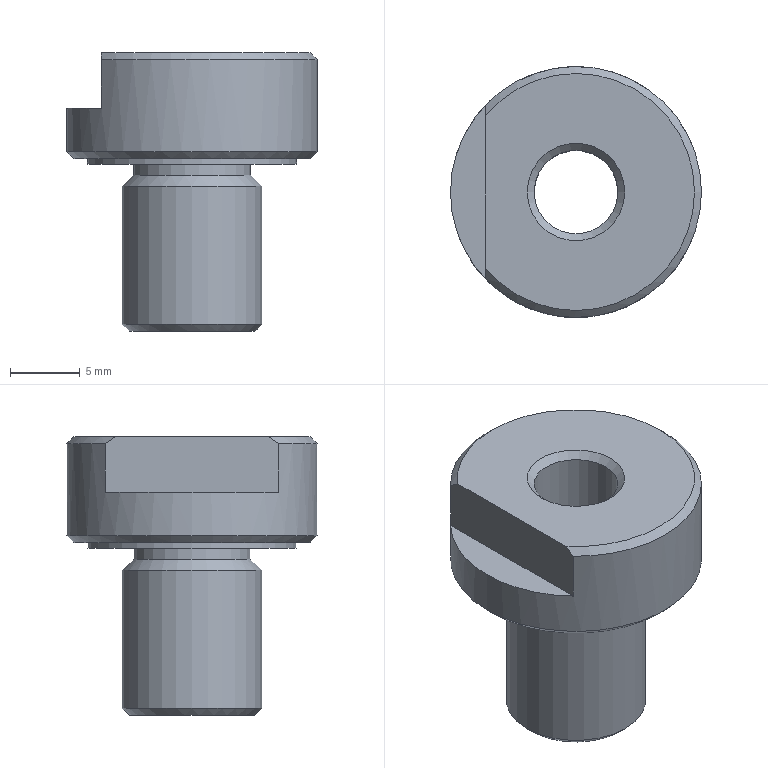Component | NX | DRILL_BUSHING | 1 solid | 17 faces | box 18 x 18 x 20 mm | volume 2247 mm3 | plane 6 | cone 6 | cylinder 5 | commonest cylinder face diameters 18 x1 15 x1 8.4 x1 10 x1 6 x1
STEP:
#1=CARTESIAN_POINT('',(0.,0.,0.));
#2=DIRECTION('',(0.,0.,1.));
#3=DIRECTION('',(1.,0.,0.));
#4=AXIS2_PLACEMENT_3D('',#1,#2,#3);
#5=CARTESIAN_POINT('',(15.5,100.638,-196.5));
#6=VERTEX_POINT('',#5);
#7=CARTESIAN_POINT('',(12.,100.638,-196.5));
#8=DIRECTION('',(0.,0.,-1.));
#9=DIRECTION('',(1.,0.,0.));
#10=AXIS2_PLACEMENT_3D('',#7,#8,#9);
#11=CIRCLE('',#10,3.5);
#12=CARTESIAN_POINT('',(12.,104.138,-196.5));
#13=DIRECTION('',(0.,0.,-1.));
#14=DIRECTION('',(1.,0.,0.));
#15=AXIS2_PLACEMENT_3D('',#12,#13,#14);
#16=PLANE('',#15);
#17=CARTESIAN_POINT('',(0.,3.5));
#18=DIRECTION('',(1.,0.));
#19=AXIS2_PLACEMENT_2D('',#17,#18);
#20=CIRCLE('',#19,3.5);
#21=(GEOMETRIC_REPRESENTATION_CONTEXT(2)PARAMETRIC_REPRESENTATION_CONTEXT()REPRESENTATION_CONTEXT('',''));
#22=DEFINITIONAL_REPRESENTATION('',(#20),#21);
#23=PCURVE('',#16,#22);
#24=CARTESIAN_POINT('',(12.,100.638,-197.));
#25=DIRECTION('',(0.,0.,1.));
#26=DIRECTION('',(-1.,0.,0.));
#27=AXIS2_PLACEMENT_3D('',#24,#25,#26);
#28=CONICAL_SURFACE('',#27,3.,0.7854);
#29=CARTESIAN_POINT('',(9.425,0.5));
#30=DIRECTION('',(-1.,0.));
#31=VECTOR('',#30,1.);
#32=LINE('',#29,#31);
#33=(GEOMETRIC_REPRESENTATION_CONTEXT(2)PARAMETRIC_REPRESENTATION_CONTEXT()REPRESENTATION_CONTEXT('',''));
#34=DEFINITIONAL_REPRESENTATION('',(#32),#33);
#35=PCURVE('',#28,#34);
#36=SURFACE_CURVE('',#11,(#23,#35),.PCURVE_S1.);
#37=EDGE_CURVE('',#6,#6,#36,.T.);
#38=ORIENTED_EDGE('',*,*,#37,.T.);
#39=EDGE_LOOP('',(#38));
#40=FACE_BOUND('',#39,.T.);
#41=CARTESIAN_POINT('',(5.5,95.161,-196.5));
#42=VERTEX_POINT('',#41);
#43=CARTESIAN_POINT('',(5.5,106.116,-196.5));
#44=VERTEX_POINT('',#43);
#45=CARTESIAN_POINT('',(5.5,88.638,-196.5));
#46=DIRECTION('',(-0.,1.,0.));
#47=VECTOR('',#46,1.);
#48=LINE('',#45,#47);
#49=CARTESIAN_POINT('',(-6.5,15.5));
#50=DIRECTION('',(-0.,-1.));
#51=VECTOR('',#50,1.);
#52=LINE('',#49,#51);
#53=(GEOMETRIC_REPRESENTATION_CONTEXT(2)PARAMETRIC_REPRESENTATION_CONTEXT()REPRESENTATION_CONTEXT('',''));
#54=DEFINITIONAL_REPRESENTATION('',(#52),#53);
#55=PCURVE('',#16,#54);
#56=CARTESIAN_POINT('',(5.5,88.638,-200.5));
#57=DIRECTION('',(1.,0.,0.));
#58=DIRECTION('',(-0.,1.,0.));
#59=AXIS2_PLACEMENT_3D('',#56,#57,#58);
#60=PLANE('',#59);
#61=CARTESIAN_POINT('',(0.,4.));
#62=DIRECTION('',(1.,0.));
#63=VECTOR('',#62,1.);
#64=LINE('',#61,#63);
#65=(GEOMETRIC_REPRESENTATION_CONTEXT(2)PARAMETRIC_REPRESENTATION_CONTEXT()REPRESENTATION_CONTEXT('',''));
#66=DEFINITIONAL_REPRESENTATION('',(#64),#65);
#67=PCURVE('',#60,#66);
#68=SURFACE_CURVE('',#48,(#55,#67),.PCURVE_S1.);
#69=EDGE_CURVE('',#42,#44,#68,.T.);
#70=ORIENTED_EDGE('',*,*,#69,.F.);
#71=CARTESIAN_POINT('',(12.,100.638,-196.5));
#72=DIRECTION('',(0.,0.,-1.));
#73=DIRECTION('',(1.,0.,0.));
#74=AXIS2_PLACEMENT_3D('',#71,#72,#73);
#75=CIRCLE('',#74,8.5);
#76=CARTESIAN_POINT('',(0.,3.5));
#77=DIRECTION('',(1.,0.));
#78=AXIS2_PLACEMENT_2D('',#76,#77);
#79=CIRCLE('',#78,8.5);
#80=(GEOMETRIC_REPRESENTATION_CONTEXT(2)PARAMETRIC_REPRESENTATION_CONTEXT()REPRESENTATION_CONTEXT('',''));
#81=DEFINITIONAL_REPRESENTATION('',(#79),#80);
#82=PCURVE('',#16,#81);
#83=CARTESIAN_POINT('',(12.,100.638,-196.5));
#84=DIRECTION('',(0.,0.,-1.));
#85=DIRECTION('',(1.,0.,0.));
#86=AXIS2_PLACEMENT_3D('',#83,#84,#85);
#87=CONICAL_SURFACE('',#86,8.5,0.7854);
#88=CARTESIAN_POINT('',(-6.283,0.));
#89=DIRECTION('',(1.,-0.));
#90=VECTOR('',#89,1.);
#91=LINE('',#88,#90);
#92=(GEOMETRIC_REPRESENTATION_CONTEXT(2)PARAMETRIC_REPRESENTATION_CONTEXT()REPRESENTATION_CONTEXT('',''));
#93=DEFINITIONAL_REPRESENTATION('',(#91),#92);
#94=PCURVE('',#87,#93);
#95=SURFACE_CURVE('',#75,(#82,#94),.PCURVE_S1.);
#96=EDGE_CURVE('',#44,#42,#95,.T.);
#97=ORIENTED_EDGE('',*,*,#96,.F.);
#98=EDGE_LOOP('',(#70,#97));
#99=FACE_BOUND('',#98,.T.);
#100=ADVANCED_FACE('',(#40,#99),#16,.F.);
#101=CARTESIAN_POINT('',(5.5,106.863,-197.));
#102=VERTEX_POINT('',#101);
#103=CARTESIAN_POINT('',(21.,100.638,-197.));
#104=VERTEX_POINT('',#103);
#105=CARTESIAN_POINT('',(12.,100.638,-197.));
#106=DIRECTION('',(0.,0.,-1.));
#107=DIRECTION('',(1.,0.,0.));
#108=AXIS2_PLACEMENT_3D('',#105,#106,#107);
#109=CIRCLE('',#108,9.);
#110=CARTESIAN_POINT('',(12.,100.638,-216.5));
#111=DIRECTION('',(0.,0.,-1.));
#112=DIRECTION('',(1.,0.,0.));
#113=AXIS2_PLACEMENT_3D('',#110,#111,#112);
#114=CYLINDRICAL_SURFACE('',#113,9.);
#115=CARTESIAN_POINT('',(0.,-19.5));
#116=DIRECTION('',(1.,0.));
#117=VECTOR('',#116,1.);
#118=LINE('',#115,#117);
#119=(GEOMETRIC_REPRESENTATION_CONTEXT(2)PARAMETRIC_REPRESENTATION_CONTEXT()REPRESENTATION_CONTEXT('',''));
#120=DEFINITIONAL_REPRESENTATION('',(#118),#119);
#121=PCURVE('',#114,#120);
#122=CARTESIAN_POINT('',(-6.283,0.5));
#123=DIRECTION('',(1.,-0.));
#124=VECTOR('',#123,1.);
#125=LINE('',#122,#124);
#126=(GEOMETRIC_REPRESENTATION_CONTEXT(2)PARAMETRIC_REPRESENTATION_CONTEXT()REPRESENTATION_CONTEXT('',''));
#127=DEFINITIONAL_REPRESENTATION('',(#125),#126);
#128=PCURVE('',#87,#127);
#129=SURFACE_CURVE('',#109,(#121,#128),.PCURVE_S1.);
#130=EDGE_CURVE('',#102,#104,#129,.T.);
#131=ORIENTED_EDGE('',*,*,#130,.T.);
#132=CARTESIAN_POINT('',(21.,100.638,-203.6));
#133=VERTEX_POINT('',#132);
#134=CARTESIAN_POINT('',(21.,100.638,-197.));
#135=CARTESIAN_POINT('',(21.,100.638,-203.6));
#136=B_SPLINE_CURVE_WITH_KNOTS('',1,(#134,#135),.UNSPECIFIED.,.F.,.F.,(2,2),(-19.5,-12.9),.PIECEWISE_BEZIER_KNOTS.);
#137=CARTESIAN_POINT('',(6.283,0.));
#138=DIRECTION('',(0.,1.));
#139=VECTOR('',#138,1.);
#140=LINE('',#137,#139);
#141=(GEOMETRIC_REPRESENTATION_CONTEXT(2)PARAMETRIC_REPRESENTATION_CONTEXT()REPRESENTATION_CONTEXT('',''));
#142=DEFINITIONAL_REPRESENTATION('',(#140),#141);
#143=PCURVE('',#114,#142);
#144=CARTESIAN_POINT('',(0.,0.));
#145=DIRECTION('',(0.,1.));
#146=VECTOR('',#145,1.);
#147=LINE('',#144,#146);
#148=(GEOMETRIC_REPRESENTATION_CONTEXT(2)PARAMETRIC_REPRESENTATION_CONTEXT()REPRESENTATION_CONTEXT('',''));
#149=DEFINITIONAL_REPRESENTATION('',(#147),#148);
#150=PCURVE('',#114,#149);
#151=SEAM_CURVE('',#136,(#143,#150),.PCURVE_S1.);
#152=EDGE_CURVE('',#104,#133,#151,.T.);
#153=ORIENTED_EDGE('',*,*,#152,.T.);
#154=CARTESIAN_POINT('',(12.,100.638,-203.6));
#155=DIRECTION('',(0.,0.,-1.));
#156=DIRECTION('',(1.,0.,0.));
#157=AXIS2_PLACEMENT_3D('',#154,#155,#156);
#158=CIRCLE('',#157,9.);
#159=CARTESIAN_POINT('',(0.,-12.9));
#160=DIRECTION('',(1.,0.));
#161=VECTOR('',#160,1.);
#162=LINE('',#159,#161);
#163=(GEOMETRIC_REPRESENTATION_CONTEXT(2)PARAMETRIC_REPRESENTATION_CONTEXT()REPRESENTATION_CONTEXT('',''));
#164=DEFINITIONAL_REPRESENTATION('',(#162),#163);
#165=PCURVE('',#114,#164);
#166=CARTESIAN_POINT('',(12.,100.638,-203.6));
#167=DIRECTION('',(0.,0.,1.));
#168=DIRECTION('',(-1.,0.,0.));
#169=AXIS2_PLACEMENT_3D('',#166,#167,#168);
#170=CONICAL_SURFACE('',#169,9.,0.7854);
#171=CARTESIAN_POINT('',(9.425,0.));
#172=DIRECTION('',(-1.,0.));
#173=VECTOR('',#172,1.);
#174=LINE('',#171,#173);
#175=(GEOMETRIC_REPRESENTATION_CONTEXT(2)PARAMETRIC_REPRESENTATION_CONTEXT()REPRESENTATION_CONTEXT('',''));
#176=DEFINITIONAL_REPRESENTATION('',(#174),#175);
#177=PCURVE('',#170,#176);
#178=SURFACE_CURVE('',#158,(#165,#177),.PCURVE_S1.);
#179=EDGE_CURVE('',#133,#133,#178,.T.);
#180=ORIENTED_EDGE('',*,*,#179,.F.);
#181=ORIENTED_EDGE('',*,*,#152,.F.);
#182=CARTESIAN_POINT('',(5.5,94.413,-197.));
#183=VERTEX_POINT('',#182);
#184=CARTESIAN_POINT('',(12.,100.638,-197.));
#185=DIRECTION('',(0.,0.,-1.));
#186=DIRECTION('',(1.,0.,0.));
#187=AXIS2_PLACEMENT_3D('',#184,#185,#186);
#188=CIRCLE('',#187,9.);
#189=CARTESIAN_POINT('',(-6.283,-19.5));
#190=DIRECTION('',(1.,0.));
#191=VECTOR('',#190,1.);
#192=LINE('',#189,#191);
#193=(GEOMETRIC_REPRESENTATION_CONTEXT(2)PARAMETRIC_REPRESENTATION_CONTEXT()REPRESENTATION_CONTEXT('',''));
#194=DEFINITIONAL_REPRESENTATION('',(#192),#193);
#195=PCURVE('',#114,#194);
#196=CARTESIAN_POINT('',(-6.283,0.5));
#197=DIRECTION('',(1.,0.));
#198=VECTOR('',#197,1.);
#199=LINE('',#196,#198);
#200=(GEOMETRIC_REPRESENTATION_CONTEXT(2)PARAMETRIC_REPRESENTATION_CONTEXT()REPRESENTATION_CONTEXT('',''));
#201=DEFINITIONAL_REPRESENTATION('',(#199),#200);
#202=PCURVE('',#87,#201);
#203=SURFACE_CURVE('',#188,(#195,#202),.PCURVE_S1.);
#204=EDGE_CURVE('',#104,#183,#203,.T.);
#205=ORIENTED_EDGE('',*,*,#204,.T.);
#206=CARTESIAN_POINT('',(5.5,94.413,-200.5));
#207=VERTEX_POINT('',#206);
#208=CARTESIAN_POINT('',(5.5,94.413,-216.5));
#209=DIRECTION('',(0.,0.,-1.));
#210=VECTOR('',#209,1.);
#211=LINE('',#208,#210);
#212=CARTESIAN_POINT('',(2.378,0.));
#213=DIRECTION('',(0.,1.));
#214=VECTOR('',#213,1.);
#215=LINE('',#212,#214);
#216=(GEOMETRIC_REPRESENTATION_CONTEXT(2)PARAMETRIC_REPRESENTATION_CONTEXT()REPRESENTATION_CONTEXT('',''));
#217=DEFINITIONAL_REPRESENTATION('',(#215),#216);
#218=PCURVE('',#114,#217);
#219=CARTESIAN_POINT('',(5.775,-16.));
#220=DIRECTION('',(0.,-1.));
#221=VECTOR('',#220,1.);
#222=LINE('',#219,#221);
#223=(GEOMETRIC_REPRESENTATION_CONTEXT(2)PARAMETRIC_REPRESENTATION_CONTEXT()REPRESENTATION_CONTEXT('',''));
#224=DEFINITIONAL_REPRESENTATION('',(#222),#223);
#225=PCURVE('',#60,#224);
#226=SURFACE_CURVE('',#211,(#218,#225),.PCURVE_S1.);
#227=EDGE_CURVE('',#183,#207,#226,.T.);
#228=ORIENTED_EDGE('',*,*,#227,.T.);
#229=CARTESIAN_POINT('',(5.5,106.863,-200.5));
#230=VERTEX_POINT('',#229);
#231=CARTESIAN_POINT('',(12.,100.638,-200.5));
#232=DIRECTION('',(0.,0.,1.));
#233=DIRECTION('',(-1.,0.,0.));
#234=AXIS2_PLACEMENT_3D('',#231,#232,#233);
#235=CIRCLE('',#234,9.);
#236=CARTESIAN_POINT('',(9.425,-16.));
#237=DIRECTION('',(-1.,0.));
#238=VECTOR('',#237,1.);
#239=LINE('',#236,#238);
#240=(GEOMETRIC_REPRESENTATION_CONTEXT(2)PARAMETRIC_REPRESENTATION_CONTEXT()REPRESENTATION_CONTEXT('',''));
#241=DEFINITIONAL_REPRESENTATION('',(#239),#240);
#242=PCURVE('',#114,#241);
#243=CARTESIAN_POINT('',(12.,100.638,-200.5));
#244=DIRECTION('',(0.,0.,1.));
#245=DIRECTION('',(-1.,0.,0.));
#246=AXIS2_PLACEMENT_3D('',#243,#244,#245);
#247=PLANE('',#246);
#248=CARTESIAN_POINT('',(0.,0.));
#249=DIRECTION('',(1.,0.));
#250=AXIS2_PLACEMENT_2D('',#248,#249);
#251=CIRCLE('',#250,9.);
#252=(GEOMETRIC_REPRESENTATION_CONTEXT(2)PARAMETRIC_REPRESENTATION_CONTEXT()REPRESENTATION_CONTEXT('',''));
#253=DEFINITIONAL_REPRESENTATION('',(#251),#252);
#254=PCURVE('',#247,#253);
#255=SURFACE_CURVE('',#235,(#242,#254),.PCURVE_S1.);
#256=EDGE_CURVE('',#230,#207,#255,.T.);
#257=ORIENTED_EDGE('',*,*,#256,.F.);
#258=CARTESIAN_POINT('',(5.5,106.863,-216.5));
#259=DIRECTION('',(0.,0.,1.));
#260=VECTOR('',#259,1.);
#261=LINE('',#258,#260);
#262=CARTESIAN_POINT('',(3.905,0.));
#263=DIRECTION('',(0.,-1.));
#264=VECTOR('',#263,1.);
#265=LINE('',#262,#264);
#266=(GEOMETRIC_REPRESENTATION_CONTEXT(2)PARAMETRIC_REPRESENTATION_CONTEXT()REPRESENTATION_CONTEXT('',''));
#267=DEFINITIONAL_REPRESENTATION('',(#265),#266);
#268=PCURVE('',#114,#267);
#269=CARTESIAN_POINT('',(18.225,-16.));
#270=DIRECTION('',(0.,1.));
#271=VECTOR('',#270,1.);
#272=LINE('',#269,#271);
#273=(GEOMETRIC_REPRESENTATION_CONTEXT(2)PARAMETRIC_REPRESENTATION_CONTEXT()REPRESENTATION_CONTEXT('',''));
#274=DEFINITIONAL_REPRESENTATION('',(#272),#273);
#275=PCURVE('',#60,#274);
#276=SURFACE_CURVE('',#261,(#268,#275),.PCURVE_S1.);
#277=EDGE_CURVE('',#230,#102,#276,.T.);
#278=ORIENTED_EDGE('',*,*,#277,.T.);
#279=EDGE_LOOP('',(#131,#153,#180,#181,#205,#228,#257,#278));
#280=FACE_BOUND('',#279,.T.);
#281=ADVANCED_FACE('',(#280),#114,.T.);
#282=CARTESIAN_POINT('',(20.5,100.638,-204.1));
#283=VERTEX_POINT('',#282);
#284=CARTESIAN_POINT('',(12.,100.638,-204.1));
#285=DIRECTION('',(0.,0.,-1.));
#286=DIRECTION('',(1.,0.,0.));
#287=AXIS2_PLACEMENT_3D('',#284,#285,#286);
#288=CIRCLE('',#287,8.5);
#289=CARTESIAN_POINT('',(9.425,-0.5));
#290=DIRECTION('',(-1.,0.));
#291=VECTOR('',#290,1.);
#292=LINE('',#289,#291);
#293=(GEOMETRIC_REPRESENTATION_CONTEXT(2)PARAMETRIC_REPRESENTATION_CONTEXT()REPRESENTATION_CONTEXT('',''));
#294=DEFINITIONAL_REPRESENTATION('',(#292),#293);
#295=PCURVE('',#170,#294);
#296=CARTESIAN_POINT('',(12.,109.138,-204.1));
#297=DIRECTION('',(0.,0.,1.));
#298=DIRECTION('',(-1.,0.,0.));
#299=AXIS2_PLACEMENT_3D('',#296,#297,#298);
#300=PLANE('',#299);
#301=CARTESIAN_POINT('',(-8.5,8.5));
#302=CARTESIAN_POINT('',(-8.5,23.222));
#303=CARTESIAN_POINT('',(4.25,15.861));
#304=CARTESIAN_POINT('',(17.,8.5));
#305=CARTESIAN_POINT('',(4.25,1.139));
#306=CARTESIAN_POINT('',(-8.5,-6.222));
#307=CARTESIAN_POINT('',(-8.5,8.5));
#308=(BOUNDED_CURVE()B_SPLINE_CURVE(2,(#301,#302,#303,#304,#305,#306,#307),.UNSPECIFIED.,.T.,.F.)B_SPLINE_CURVE_WITH_KNOTS((1,2,2,2,2,1),(-2.094,0.,2.094,4.189,6.283,8.378),.UNSPECIFIED.)CURVE()GEOMETRIC_REPRESENTATION_ITEM()RATIONAL_B_SPLINE_CURVE((1.,0.5,1.,0.5,1.,0.5,1.))REPRESENTATION_ITEM(''));
#309=(GEOMETRIC_REPRESENTATION_CONTEXT(2)PARAMETRIC_REPRESENTATION_CONTEXT()REPRESENTATION_CONTEXT('',''));
#310=DEFINITIONAL_REPRESENTATION('',(#308),#309);
#311=PCURVE('',#300,#310);
#312=SURFACE_CURVE('',#288,(#295,#311),.PCURVE_S1.);
#313=EDGE_CURVE('',#283,#283,#312,.T.);
#314=ORIENTED_EDGE('',*,*,#313,.F.);
#315=CARTESIAN_POINT('',(20.5,100.638,-204.1));
#316=CARTESIAN_POINT('',(21.,100.638,-203.6));
#317=B_SPLINE_CURVE_WITH_KNOTS('',1,(#315,#316),.UNSPECIFIED.,.F.,.F.,(2,2),(-0.7071,0.),.PIECEWISE_BEZIER_KNOTS.);
#318=CARTESIAN_POINT('',(9.425,0.));
#319=DIRECTION('',(0.,1.));
#320=VECTOR('',#319,1.);
#321=LINE('',#318,#320);
#322=(GEOMETRIC_REPRESENTATION_CONTEXT(2)PARAMETRIC_REPRESENTATION_CONTEXT()REPRESENTATION_CONTEXT('',''));
#323=DEFINITIONAL_REPRESENTATION('',(#321),#322);
#324=PCURVE('',#170,#323);
#325=CARTESIAN_POINT('',(3.142,0.));
#326=DIRECTION('',(0.,1.));
#327=VECTOR('',#326,1.);
#328=LINE('',#325,#327);
#329=(GEOMETRIC_REPRESENTATION_CONTEXT(2)PARAMETRIC_REPRESENTATION_CONTEXT()REPRESENTATION_CONTEXT('',''));
#330=DEFINITIONAL_REPRESENTATION('',(#328),#329);
#331=PCURVE('',#170,#330);
#332=SEAM_CURVE('',#317,(#324,#331),.PCURVE_S1.);
#333=EDGE_CURVE('',#283,#133,#332,.T.);
#334=ORIENTED_EDGE('',*,*,#333,.T.);
#335=ORIENTED_EDGE('',*,*,#179,.T.);
#336=ORIENTED_EDGE('',*,*,#333,.F.);
#337=EDGE_LOOP('',(#314,#334,#335,#336));
#338=FACE_BOUND('',#337,.T.);
#339=ADVANCED_FACE('',(#338),#170,.T.);
#340=CARTESIAN_POINT('',(19.5,100.638,-204.1));
#341=VERTEX_POINT('',#340);
#342=CARTESIAN_POINT('',(12.,100.638,-204.1));
#343=DIRECTION('',(0.,0.,-1.));
#344=DIRECTION('',(1.,0.,0.));
#345=AXIS2_PLACEMENT_3D('',#342,#343,#344);
#346=CIRCLE('',#345,7.5);
#347=CARTESIAN_POINT('',(-7.5,8.5));
#348=CARTESIAN_POINT('',(-7.5,21.49));
#349=CARTESIAN_POINT('',(3.75,14.995));
#350=CARTESIAN_POINT('',(15.,8.5));
#351=CARTESIAN_POINT('',(3.75,2.005));
#352=CARTESIAN_POINT('',(-7.5,-4.49));
#353=CARTESIAN_POINT('',(-7.5,8.5));
#354=(BOUNDED_CURVE()B_SPLINE_CURVE(2,(#347,#348,#349,#350,#351,#352,#353),.UNSPECIFIED.,.T.,.F.)B_SPLINE_CURVE_WITH_KNOTS((1,2,2,2,2,1),(-2.094,0.,2.094,4.189,6.283,8.378),.UNSPECIFIED.)CURVE()GEOMETRIC_REPRESENTATION_ITEM()RATIONAL_B_SPLINE_CURVE((1.,0.5,1.,0.5,1.,0.5,1.))REPRESENTATION_ITEM(''));
#355=(GEOMETRIC_REPRESENTATION_CONTEXT(2)PARAMETRIC_REPRESENTATION_CONTEXT()REPRESENTATION_CONTEXT('',''));
#356=DEFINITIONAL_REPRESENTATION('',(#354),#355);
#357=PCURVE('',#300,#356);
#358=CARTESIAN_POINT('',(12.,100.638,-216.5));
#359=DIRECTION('',(0.,0.,-1.));
#360=DIRECTION('',(1.,0.,0.));
#361=AXIS2_PLACEMENT_3D('',#358,#359,#360);
#362=CYLINDRICAL_SURFACE('',#361,7.5);
#363=CARTESIAN_POINT('',(0.,-12.4));
#364=DIRECTION('',(1.,0.));
#365=VECTOR('',#364,1.);
#366=LINE('',#363,#365);
#367=(GEOMETRIC_REPRESENTATION_CONTEXT(2)PARAMETRIC_REPRESENTATION_CONTEXT()REPRESENTATION_CONTEXT('',''));
#368=DEFINITIONAL_REPRESENTATION('',(#366),#367);
#369=PCURVE('',#362,#368);
#370=SURFACE_CURVE('',#346,(#357,#369),.PCURVE_S1.);
#371=EDGE_CURVE('',#341,#341,#370,.T.);
#372=ORIENTED_EDGE('',*,*,#371,.F.);
#373=EDGE_LOOP('',(#372));
#374=FACE_BOUND('',#373,.T.);
#375=ORIENTED_EDGE('',*,*,#313,.T.);
#376=EDGE_LOOP('',(#375));
#377=FACE_BOUND('',#376,.T.);
#378=ADVANCED_FACE('',(#374,#377),#300,.F.);
#379=CARTESIAN_POINT('',(19.5,100.638,-204.5));
#380=VERTEX_POINT('',#379);
#381=CARTESIAN_POINT('',(12.,100.638,-204.5));
#382=DIRECTION('',(0.,0.,-1.));
#383=DIRECTION('',(1.,0.,0.));
#384=AXIS2_PLACEMENT_3D('',#381,#382,#383);
#385=CIRCLE('',#384,7.5);
#386=CARTESIAN_POINT('',(0.,-12.));
#387=DIRECTION('',(1.,0.));
#388=VECTOR('',#387,1.);
#389=LINE('',#386,#388);
#390=(GEOMETRIC_REPRESENTATION_CONTEXT(2)PARAMETRIC_REPRESENTATION_CONTEXT()REPRESENTATION_CONTEXT('',''));
#391=DEFINITIONAL_REPRESENTATION('',(#389),#390);
#392=PCURVE('',#362,#391);
#393=CARTESIAN_POINT('',(12.,108.138,-204.5));
#394=DIRECTION('',(0.,0.,1.));
#395=DIRECTION('',(-1.,0.,0.));
#396=AXIS2_PLACEMENT_3D('',#393,#394,#395);
#397=PLANE('',#396);
#398=CARTESIAN_POINT('',(-7.5,7.5));
#399=CARTESIAN_POINT('',(-7.5,20.49));
#400=CARTESIAN_POINT('',(3.75,13.995));
#401=CARTESIAN_POINT('',(15.,7.5));
#402=CARTESIAN_POINT('',(3.75,1.005));
#403=CARTESIAN_POINT('',(-7.5,-5.49));
#404=CARTESIAN_POINT('',(-7.5,7.5));
#405=(BOUNDED_CURVE()B_SPLINE_CURVE(2,(#398,#399,#400,#401,#402,#403,#404),.UNSPECIFIED.,.T.,.F.)B_SPLINE_CURVE_WITH_KNOTS((1,2,2,2,2,1),(-2.094,0.,2.094,4.189,6.283,8.378),.UNSPECIFIED.)CURVE()GEOMETRIC_REPRESENTATION_ITEM()RATIONAL_B_SPLINE_CURVE((1.,0.5,1.,0.5,1.,0.5,1.))REPRESENTATION_ITEM(''));
#406=(GEOMETRIC_REPRESENTATION_CONTEXT(2)PARAMETRIC_REPRESENTATION_CONTEXT()REPRESENTATION_CONTEXT('',''));
#407=DEFINITIONAL_REPRESENTATION('',(#405),#406);
#408=PCURVE('',#397,#407);
#409=SURFACE_CURVE('',#385,(#392,#408),.PCURVE_S1.);
#410=EDGE_CURVE('',#380,#380,#409,.T.);
#411=ORIENTED_EDGE('',*,*,#410,.F.);
#412=CARTESIAN_POINT('',(19.5,100.638,-204.1));
#413=CARTESIAN_POINT('',(19.5,100.638,-204.5));
#414=B_SPLINE_CURVE_WITH_KNOTS('',1,(#412,#413),.UNSPECIFIED.,.F.,.F.,(2,2),(-12.4,-12.),.PIECEWISE_BEZIER_KNOTS.);
#415=CARTESIAN_POINT('',(0.,0.));
#416=DIRECTION('',(0.,1.));
#417=VECTOR('',#416,1.);
#418=LINE('',#415,#417);
#419=(GEOMETRIC_REPRESENTATION_CONTEXT(2)PARAMETRIC_REPRESENTATION_CONTEXT()REPRESENTATION_CONTEXT('',''));
#420=DEFINITIONAL_REPRESENTATION('',(#418),#419);
#421=PCURVE('',#362,#420);
#422=CARTESIAN_POINT('',(6.283,0.));
#423=DIRECTION('',(0.,1.));
#424=VECTOR('',#423,1.);
#425=LINE('',#422,#424);
#426=(GEOMETRIC_REPRESENTATION_CONTEXT(2)PARAMETRIC_REPRESENTATION_CONTEXT()REPRESENTATION_CONTEXT('',''));
#427=DEFINITIONAL_REPRESENTATION('',(#425),#426);
#428=PCURVE('',#362,#427);
#429=SEAM_CURVE('',#414,(#421,#428),.PCURVE_S1.);
#430=EDGE_CURVE('',#341,#380,#429,.T.);
#431=ORIENTED_EDGE('',*,*,#430,.F.);
#432=ORIENTED_EDGE('',*,*,#371,.T.);
#433=ORIENTED_EDGE('',*,*,#430,.T.);
#434=EDGE_LOOP('',(#411,#431,#432,#433));
#435=FACE_BOUND('',#434,.T.);
#436=ADVANCED_FACE('',(#435),#362,.T.);
#437=CARTESIAN_POINT('',(16.2,100.638,-204.5));
#438=VERTEX_POINT('',#437);
#439=CARTESIAN_POINT('',(12.,100.638,-204.5));
#440=DIRECTION('',(0.,0.,-1.));
#441=DIRECTION('',(1.,0.,0.));
#442=AXIS2_PLACEMENT_3D('',#439,#440,#441);
#443=CIRCLE('',#442,4.2);
#444=CARTESIAN_POINT('',(-4.2,7.5));
#445=CARTESIAN_POINT('',(-4.2,14.775));
#446=CARTESIAN_POINT('',(2.1,11.137));
#447=CARTESIAN_POINT('',(8.4,7.5));
#448=CARTESIAN_POINT('',(2.1,3.863));
#449=CARTESIAN_POINT('',(-4.2,0.2254));
#450=CARTESIAN_POINT('',(-4.2,7.5));
#451=(BOUNDED_CURVE()B_SPLINE_CURVE(2,(#444,#445,#446,#447,#448,#449,#450),.UNSPECIFIED.,.T.,.F.)B_SPLINE_CURVE_WITH_KNOTS((1,2,2,2,2,1),(-2.094,0.,2.094,4.189,6.283,8.378),.UNSPECIFIED.)CURVE()GEOMETRIC_REPRESENTATION_ITEM()RATIONAL_B_SPLINE_CURVE((1.,0.5,1.,0.5,1.,0.5,1.))REPRESENTATION_ITEM(''));
#452=(GEOMETRIC_REPRESENTATION_CONTEXT(2)PARAMETRIC_REPRESENTATION_CONTEXT()REPRESENTATION_CONTEXT('',''));
#453=DEFINITIONAL_REPRESENTATION('',(#451),#452);
#454=PCURVE('',#397,#453);
#455=CARTESIAN_POINT('',(12.,100.638,-216.5));
#456=DIRECTION('',(0.,0.,-1.));
#457=DIRECTION('',(1.,0.,0.));
#458=AXIS2_PLACEMENT_3D('',#455,#456,#457);
#459=CYLINDRICAL_SURFACE('',#458,4.2);
#460=CARTESIAN_POINT('',(0.,-12.));
#461=DIRECTION('',(1.,0.));
#462=VECTOR('',#461,1.);
#463=LINE('',#460,#462);
#464=(GEOMETRIC_REPRESENTATION_CONTEXT(2)PARAMETRIC_REPRESENTATION_CONTEXT()REPRESENTATION_CONTEXT('',''));
#465=DEFINITIONAL_REPRESENTATION('',(#463),#464);
#466=PCURVE('',#459,#465);
#467=SURFACE_CURVE('',#443,(#454,#466),.PCURVE_S1.);
#468=EDGE_CURVE('',#438,#438,#467,.T.);
#469=ORIENTED_EDGE('',*,*,#468,.F.);
#470=EDGE_LOOP('',(#469));
#471=FACE_BOUND('',#470,.T.);
#472=ORIENTED_EDGE('',*,*,#410,.T.);
#473=EDGE_LOOP('',(#472));
#474=FACE_BOUND('',#473,.T.);
#475=ADVANCED_FACE('',(#471,#474),#397,.F.);
#476=CARTESIAN_POINT('',(16.2,100.638,-205.3));
#477=VERTEX_POINT('',#476);
#478=CARTESIAN_POINT('',(12.,100.638,-205.3));
#479=DIRECTION('',(0.,0.,-1.));
#480=DIRECTION('',(1.,0.,0.));
#481=AXIS2_PLACEMENT_3D('',#478,#479,#480);
#482=CIRCLE('',#481,4.2);
#483=CARTESIAN_POINT('',(0.,-11.2));
#484=DIRECTION('',(1.,0.));
#485=VECTOR('',#484,1.);
#486=LINE('',#483,#485);
#487=(GEOMETRIC_REPRESENTATION_CONTEXT(2)PARAMETRIC_REPRESENTATION_CONTEXT()REPRESENTATION_CONTEXT('',''));
#488=DEFINITIONAL_REPRESENTATION('',(#486),#487);
#489=PCURVE('',#459,#488);
#490=CARTESIAN_POINT('',(12.,100.638,-205.3));
#491=DIRECTION('',(0.,0.,-1.));
#492=DIRECTION('',(1.,0.,0.));
#493=AXIS2_PLACEMENT_3D('',#490,#491,#492);
#494=CONICAL_SURFACE('',#493,4.2,0.7854);
#495=CARTESIAN_POINT('',(0.,-0.));
#496=DIRECTION('',(1.,0.));
#497=VECTOR('',#496,1.);
#498=LINE('',#495,#497);
#499=(GEOMETRIC_REPRESENTATION_CONTEXT(2)PARAMETRIC_REPRESENTATION_CONTEXT()REPRESENTATION_CONTEXT('',''));
#500=DEFINITIONAL_REPRESENTATION('',(#498),#499);
#501=PCURVE('',#494,#500);
#502=SURFACE_CURVE('',#482,(#489,#501),.PCURVE_S1.);
#503=EDGE_CURVE('',#477,#477,#502,.T.);
#504=ORIENTED_EDGE('',*,*,#503,.F.);
#505=CARTESIAN_POINT('',(16.2,100.638,-204.5));
#506=CARTESIAN_POINT('',(16.2,100.638,-205.3));
#507=B_SPLINE_CURVE_WITH_KNOTS('',1,(#505,#506),.UNSPECIFIED.,.F.,.F.,(2,2),(-12.,-11.2),.PIECEWISE_BEZIER_KNOTS.);
#508=CARTESIAN_POINT('',(0.,0.));
#509=DIRECTION('',(0.,1.));
#510=VECTOR('',#509,1.);
#511=LINE('',#508,#510);
#512=(GEOMETRIC_REPRESENTATION_CONTEXT(2)PARAMETRIC_REPRESENTATION_CONTEXT()REPRESENTATION_CONTEXT('',''));
#513=DEFINITIONAL_REPRESENTATION('',(#511),#512);
#514=PCURVE('',#459,#513);
#515=CARTESIAN_POINT('',(6.283,0.));
#516=DIRECTION('',(0.,1.));
#517=VECTOR('',#516,1.);
#518=LINE('',#515,#517);
#519=(GEOMETRIC_REPRESENTATION_CONTEXT(2)PARAMETRIC_REPRESENTATION_CONTEXT()REPRESENTATION_CONTEXT('',''));
#520=DEFINITIONAL_REPRESENTATION('',(#518),#519);
#521=PCURVE('',#459,#520);
#522=SEAM_CURVE('',#507,(#514,#521),.PCURVE_S1.);
#523=EDGE_CURVE('',#438,#477,#522,.T.);
#524=ORIENTED_EDGE('',*,*,#523,.F.);
#525=ORIENTED_EDGE('',*,*,#468,.T.);
#526=ORIENTED_EDGE('',*,*,#523,.T.);
#527=EDGE_LOOP('',(#504,#524,#525,#526));
#528=FACE_BOUND('',#527,.T.);
#529=ADVANCED_FACE('',(#528),#459,.T.);
#530=CARTESIAN_POINT('',(17.,100.638,-206.1));
#531=VERTEX_POINT('',#530);
#532=CARTESIAN_POINT('',(12.,100.638,-206.1));
#533=DIRECTION('',(0.,0.,-1.));
#534=DIRECTION('',(1.,0.,0.));
#535=AXIS2_PLACEMENT_3D('',#532,#533,#534);
#536=CIRCLE('',#535,5.);
#537=CARTESIAN_POINT('',(0.,0.8));
#538=DIRECTION('',(1.,0.));
#539=VECTOR('',#538,1.);
#540=LINE('',#537,#539);
#541=(GEOMETRIC_REPRESENTATION_CONTEXT(2)PARAMETRIC_REPRESENTATION_CONTEXT()REPRESENTATION_CONTEXT('',''));
#542=DEFINITIONAL_REPRESENTATION('',(#540),#541);
#543=PCURVE('',#494,#542);
#544=CARTESIAN_POINT('',(12.,100.638,-216.5));
#545=DIRECTION('',(0.,0.,-1.));
#546=DIRECTION('',(1.,0.,0.));
#547=AXIS2_PLACEMENT_3D('',#544,#545,#546);
#548=CYLINDRICAL_SURFACE('',#547,5.);
#549=CARTESIAN_POINT('',(0.,-10.4));
#550=DIRECTION('',(1.,0.));
#551=VECTOR('',#550,1.);
#552=LINE('',#549,#551);
#553=(GEOMETRIC_REPRESENTATION_CONTEXT(2)PARAMETRIC_REPRESENTATION_CONTEXT()REPRESENTATION_CONTEXT('',''));
#554=DEFINITIONAL_REPRESENTATION('',(#552),#553);
#555=PCURVE('',#548,#554);
#556=SURFACE_CURVE('',#536,(#543,#555),.PCURVE_S1.);
#557=EDGE_CURVE('',#531,#531,#556,.T.);
#558=ORIENTED_EDGE('',*,*,#557,.F.);
#559=CARTESIAN_POINT('',(16.2,100.638,-205.3));
#560=CARTESIAN_POINT('',(17.,100.638,-206.1));
#561=B_SPLINE_CURVE_WITH_KNOTS('',1,(#559,#560),.UNSPECIFIED.,.F.,.F.,(2,2),(-0.,1.131),.PIECEWISE_BEZIER_KNOTS.);
#562=CARTESIAN_POINT('',(0.,0.));
#563=DIRECTION('',(0.,1.));
#564=VECTOR('',#563,1.);
#565=LINE('',#562,#564);
#566=(GEOMETRIC_REPRESENTATION_CONTEXT(2)PARAMETRIC_REPRESENTATION_CONTEXT()REPRESENTATION_CONTEXT('',''));
#567=DEFINITIONAL_REPRESENTATION('',(#565),#566);
#568=PCURVE('',#494,#567);
#569=CARTESIAN_POINT('',(6.283,0.));
#570=DIRECTION('',(0.,1.));
#571=VECTOR('',#570,1.);
#572=LINE('',#569,#571);
#573=(GEOMETRIC_REPRESENTATION_CONTEXT(2)PARAMETRIC_REPRESENTATION_CONTEXT()REPRESENTATION_CONTEXT('',''));
#574=DEFINITIONAL_REPRESENTATION('',(#572),#573);
#575=PCURVE('',#494,#574);
#576=SEAM_CURVE('',#561,(#568,#575),.PCURVE_S1.);
#577=EDGE_CURVE('',#477,#531,#576,.T.);
#578=ORIENTED_EDGE('',*,*,#577,.F.);
#579=ORIENTED_EDGE('',*,*,#503,.T.);
#580=ORIENTED_EDGE('',*,*,#577,.T.);
#581=EDGE_LOOP('',(#558,#578,#579,#580));
#582=FACE_BOUND('',#581,.T.);
#583=ADVANCED_FACE('',(#582),#494,.T.);
#584=CARTESIAN_POINT('',(17.,100.638,-216.));
#585=VERTEX_POINT('',#584);
#586=CARTESIAN_POINT('',(12.,100.638,-216.));
#587=DIRECTION('',(0.,0.,-1.));
#588=DIRECTION('',(1.,0.,0.));
#589=AXIS2_PLACEMENT_3D('',#586,#587,#588);
#590=CIRCLE('',#589,5.);
#591=CARTESIAN_POINT('',(0.,-0.5));
#592=DIRECTION('',(1.,0.));
#593=VECTOR('',#592,1.);
#594=LINE('',#591,#593);
#595=(GEOMETRIC_REPRESENTATION_CONTEXT(2)PARAMETRIC_REPRESENTATION_CONTEXT()REPRESENTATION_CONTEXT('',''));
#596=DEFINITIONAL_REPRESENTATION('',(#594),#595);
#597=PCURVE('',#548,#596);
#598=CARTESIAN_POINT('',(12.,100.638,-216.));
#599=DIRECTION('',(0.,0.,1.));
#600=DIRECTION('',(-1.,0.,0.));
#601=AXIS2_PLACEMENT_3D('',#598,#599,#600);
#602=CONICAL_SURFACE('',#601,5.,0.7854);
#603=CARTESIAN_POINT('',(9.425,0.));
#604=DIRECTION('',(-1.,0.));
#605=VECTOR('',#604,1.);
#606=LINE('',#603,#605);
#607=(GEOMETRIC_REPRESENTATION_CONTEXT(2)PARAMETRIC_REPRESENTATION_CONTEXT()REPRESENTATION_CONTEXT('',''));
#608=DEFINITIONAL_REPRESENTATION('',(#606),#607);
#609=PCURVE('',#602,#608);
#610=SURFACE_CURVE('',#590,(#597,#609),.PCURVE_S1.);
#611=EDGE_CURVE('',#585,#585,#610,.T.);
#612=ORIENTED_EDGE('',*,*,#611,.F.);
#613=CARTESIAN_POINT('',(17.,100.638,-206.1));
#614=CARTESIAN_POINT('',(17.,100.638,-216.));
#615=B_SPLINE_CURVE_WITH_KNOTS('',1,(#613,#614),.UNSPECIFIED.,.F.,.F.,(2,2),(-10.4,-0.5),.PIECEWISE_BEZIER_KNOTS.);
#616=CARTESIAN_POINT('',(0.,0.));
#617=DIRECTION('',(0.,1.));
#618=VECTOR('',#617,1.);
#619=LINE('',#616,#618);
#620=(GEOMETRIC_REPRESENTATION_CONTEXT(2)PARAMETRIC_REPRESENTATION_CONTEXT()REPRESENTATION_CONTEXT('',''));
#621=DEFINITIONAL_REPRESENTATION('',(#619),#620);
#622=PCURVE('',#548,#621);
#623=CARTESIAN_POINT('',(6.283,0.));
#624=DIRECTION('',(0.,1.));
#625=VECTOR('',#624,1.);
#626=LINE('',#623,#625);
#627=(GEOMETRIC_REPRESENTATION_CONTEXT(2)PARAMETRIC_REPRESENTATION_CONTEXT()REPRESENTATION_CONTEXT('',''));
#628=DEFINITIONAL_REPRESENTATION('',(#626),#627);
#629=PCURVE('',#548,#628);
#630=SEAM_CURVE('',#615,(#622,#629),.PCURVE_S1.);
#631=EDGE_CURVE('',#531,#585,#630,.T.);
#632=ORIENTED_EDGE('',*,*,#631,.F.);
#633=ORIENTED_EDGE('',*,*,#557,.T.);
#634=ORIENTED_EDGE('',*,*,#631,.T.);
#635=EDGE_LOOP('',(#612,#632,#633,#634));
#636=FACE_BOUND('',#635,.T.);
#637=ADVANCED_FACE('',(#636),#548,.T.);
#638=CARTESIAN_POINT('',(16.5,100.638,-216.5));
#639=VERTEX_POINT('',#638);
#640=CARTESIAN_POINT('',(12.,100.638,-216.5));
#641=DIRECTION('',(0.,0.,-1.));
#642=DIRECTION('',(1.,0.,0.));
#643=AXIS2_PLACEMENT_3D('',#640,#641,#642);
#644=CIRCLE('',#643,4.5);
#645=CARTESIAN_POINT('',(9.425,-0.5));
#646=DIRECTION('',(-1.,0.));
#647=VECTOR('',#646,1.);
#648=LINE('',#645,#647);
#649=(GEOMETRIC_REPRESENTATION_CONTEXT(2)PARAMETRIC_REPRESENTATION_CONTEXT()REPRESENTATION_CONTEXT('',''));
#650=DEFINITIONAL_REPRESENTATION('',(#648),#649);
#651=PCURVE('',#602,#650);
#652=CARTESIAN_POINT('',(12.,105.138,-216.5));
#653=DIRECTION('',(0.,0.,1.));
#654=DIRECTION('',(-1.,0.,0.));
#655=AXIS2_PLACEMENT_3D('',#652,#653,#654);
#656=PLANE('',#655);
#657=CARTESIAN_POINT('',(-4.5,4.5));
#658=CARTESIAN_POINT('',(-4.5,12.294));
#659=CARTESIAN_POINT('',(2.25,8.397));
#660=CARTESIAN_POINT('',(9.,4.5));
#661=CARTESIAN_POINT('',(2.25,0.6029));
#662=CARTESIAN_POINT('',(-4.5,-3.294));
#663=CARTESIAN_POINT('',(-4.5,4.5));
#664=(BOUNDED_CURVE()B_SPLINE_CURVE(2,(#657,#658,#659,#660,#661,#662,#663),.UNSPECIFIED.,.T.,.F.)B_SPLINE_CURVE_WITH_KNOTS((1,2,2,2,2,1),(-2.094,0.,2.094,4.189,6.283,8.378),.UNSPECIFIED.)CURVE()GEOMETRIC_REPRESENTATION_ITEM()RATIONAL_B_SPLINE_CURVE((1.,0.5,1.,0.5,1.,0.5,1.))REPRESENTATION_ITEM(''));
#665=(GEOMETRIC_REPRESENTATION_CONTEXT(2)PARAMETRIC_REPRESENTATION_CONTEXT()REPRESENTATION_CONTEXT('',''));
#666=DEFINITIONAL_REPRESENTATION('',(#664),#665);
#667=PCURVE('',#656,#666);
#668=SURFACE_CURVE('',#644,(#651,#667),.PCURVE_S1.);
#669=EDGE_CURVE('',#639,#639,#668,.T.);
#670=ORIENTED_EDGE('',*,*,#669,.F.);
#671=CARTESIAN_POINT('',(16.5,100.638,-216.5));
#672=CARTESIAN_POINT('',(17.,100.638,-216.));
#673=B_SPLINE_CURVE_WITH_KNOTS('',1,(#671,#672),.UNSPECIFIED.,.F.,.F.,(2,2),(-0.7071,0.),.PIECEWISE_BEZIER_KNOTS.);
#674=CARTESIAN_POINT('',(9.425,0.));
#675=DIRECTION('',(0.,1.));
#676=VECTOR('',#675,1.);
#677=LINE('',#674,#676);
#678=(GEOMETRIC_REPRESENTATION_CONTEXT(2)PARAMETRIC_REPRESENTATION_CONTEXT()REPRESENTATION_CONTEXT('',''));
#679=DEFINITIONAL_REPRESENTATION('',(#677),#678);
#680=PCURVE('',#602,#679);
#681=CARTESIAN_POINT('',(3.142,0.));
#682=DIRECTION('',(0.,1.));
#683=VECTOR('',#682,1.);
#684=LINE('',#681,#683);
#685=(GEOMETRIC_REPRESENTATION_CONTEXT(2)PARAMETRIC_REPRESENTATION_CONTEXT()REPRESENTATION_CONTEXT('',''));
#686=DEFINITIONAL_REPRESENTATION('',(#684),#685);
#687=PCURVE('',#602,#686);
#688=SEAM_CURVE('',#673,(#680,#687),.PCURVE_S1.);
#689=EDGE_CURVE('',#639,#585,#688,.T.);
#690=ORIENTED_EDGE('',*,*,#689,.T.);
#691=ORIENTED_EDGE('',*,*,#611,.T.);
#692=ORIENTED_EDGE('',*,*,#689,.F.);
#693=EDGE_LOOP('',(#670,#690,#691,#692));
#694=FACE_BOUND('',#693,.T.);
#695=ADVANCED_FACE('',(#694),#602,.T.);
#696=CARTESIAN_POINT('',(15.5,100.638,-216.5));
#697=VERTEX_POINT('',#696);
#698=CARTESIAN_POINT('',(12.,100.638,-216.5));
#699=DIRECTION('',(0.,0.,-1.));
#700=DIRECTION('',(1.,0.,0.));
#701=AXIS2_PLACEMENT_3D('',#698,#699,#700);
#702=CIRCLE('',#701,3.5);
#703=CARTESIAN_POINT('',(-3.5,4.5));
#704=CARTESIAN_POINT('',(-3.5,10.562));
#705=CARTESIAN_POINT('',(1.75,7.531));
#706=CARTESIAN_POINT('',(7.,4.5));
#707=CARTESIAN_POINT('',(1.75,1.469));
#708=CARTESIAN_POINT('',(-3.5,-1.562));
#709=CARTESIAN_POINT('',(-3.5,4.5));
#710=(BOUNDED_CURVE()B_SPLINE_CURVE(2,(#703,#704,#705,#706,#707,#708,#709),.UNSPECIFIED.,.T.,.F.)B_SPLINE_CURVE_WITH_KNOTS((1,2,2,2,2,1),(-2.094,0.,2.094,4.189,6.283,8.378),.UNSPECIFIED.)CURVE()GEOMETRIC_REPRESENTATION_ITEM()RATIONAL_B_SPLINE_CURVE((1.,0.5,1.,0.5,1.,0.5,1.))REPRESENTATION_ITEM(''));
#711=(GEOMETRIC_REPRESENTATION_CONTEXT(2)PARAMETRIC_REPRESENTATION_CONTEXT()REPRESENTATION_CONTEXT('',''));
#712=DEFINITIONAL_REPRESENTATION('',(#710),#711);
#713=PCURVE('',#656,#712);
#714=CARTESIAN_POINT('',(12.,100.638,-216.5));
#715=DIRECTION('',(0.,0.,-1.));
#716=DIRECTION('',(1.,0.,0.));
#717=AXIS2_PLACEMENT_3D('',#714,#715,#716);
#718=CONICAL_SURFACE('',#717,3.5,0.7854);
#719=CARTESIAN_POINT('',(0.,0.));
#720=DIRECTION('',(1.,0.));
#721=VECTOR('',#720,1.);
#722=LINE('',#719,#721);
#723=(GEOMETRIC_REPRESENTATION_CONTEXT(2)PARAMETRIC_REPRESENTATION_CONTEXT()REPRESENTATION_CONTEXT('',''));
#724=DEFINITIONAL_REPRESENTATION('',(#722),#723);
#725=PCURVE('',#718,#724);
#726=SURFACE_CURVE('',#702,(#713,#725),.PCURVE_S1.);
#727=EDGE_CURVE('',#697,#697,#726,.T.);
#728=ORIENTED_EDGE('',*,*,#727,.F.);
#729=EDGE_LOOP('',(#728));
#730=FACE_BOUND('',#729,.T.);
#731=ORIENTED_EDGE('',*,*,#669,.T.);
#732=EDGE_LOOP('',(#731));
#733=FACE_BOUND('',#732,.T.);
#734=ADVANCED_FACE('',(#730,#733),#656,.F.);
#735=CARTESIAN_POINT('',(15.,100.638,-216.));
#736=VERTEX_POINT('',#735);
#737=CARTESIAN_POINT('',(12.,100.638,-216.));
#738=DIRECTION('',(0.,0.,-1.));
#739=DIRECTION('',(1.,0.,0.));
#740=AXIS2_PLACEMENT_3D('',#737,#738,#739);
#741=CIRCLE('',#740,3.);
#742=CARTESIAN_POINT('',(0.,-0.5));
#743=DIRECTION('',(1.,0.));
#744=VECTOR('',#743,1.);
#745=LINE('',#742,#744);
#746=(GEOMETRIC_REPRESENTATION_CONTEXT(2)PARAMETRIC_REPRESENTATION_CONTEXT()REPRESENTATION_CONTEXT('',''));
#747=DEFINITIONAL_REPRESENTATION('',(#745),#746);
#748=PCURVE('',#718,#747);
#749=CARTESIAN_POINT('',(12.,100.638,-216.5));
#750=DIRECTION('',(0.,0.,-1.));
#751=DIRECTION('',(1.,0.,0.));
#752=AXIS2_PLACEMENT_3D('',#749,#750,#751);
#753=CYLINDRICAL_SURFACE('',#752,3.);
#754=CARTESIAN_POINT('',(0.,-0.5));
#755=DIRECTION('',(1.,0.));
#756=VECTOR('',#755,1.);
#757=LINE('',#754,#756);
#758=(GEOMETRIC_REPRESENTATION_CONTEXT(2)PARAMETRIC_REPRESENTATION_CONTEXT()REPRESENTATION_CONTEXT('',''));
#759=DEFINITIONAL_REPRESENTATION('',(#757),#758);
#760=PCURVE('',#753,#759);
#761=SURFACE_CURVE('',#741,(#748,#760),.PCURVE_S1.);
#762=EDGE_CURVE('',#736,#736,#761,.T.);
#763=ORIENTED_EDGE('',*,*,#762,.T.);
#764=CARTESIAN_POINT('',(15.,100.638,-216.));
#765=CARTESIAN_POINT('',(15.5,100.638,-216.5));
#766=B_SPLINE_CURVE_WITH_KNOTS('',1,(#764,#765),.UNSPECIFIED.,.F.,.F.,(2,2),(-0.7071,0.),.PIECEWISE_BEZIER_KNOTS.);
#767=CARTESIAN_POINT('',(6.283,0.));
#768=DIRECTION('',(0.,1.));
#769=VECTOR('',#768,1.);
#770=LINE('',#767,#769);
#771=(GEOMETRIC_REPRESENTATION_CONTEXT(2)PARAMETRIC_REPRESENTATION_CONTEXT()REPRESENTATION_CONTEXT('',''));
#772=DEFINITIONAL_REPRESENTATION('',(#770),#771);
#773=PCURVE('',#718,#772);
#774=CARTESIAN_POINT('',(0.,0.));
#775=DIRECTION('',(0.,1.));
#776=VECTOR('',#775,1.);
#777=LINE('',#774,#776);
#778=(GEOMETRIC_REPRESENTATION_CONTEXT(2)PARAMETRIC_REPRESENTATION_CONTEXT()REPRESENTATION_CONTEXT('',''));
#779=DEFINITIONAL_REPRESENTATION('',(#777),#778);
#780=PCURVE('',#718,#779);
#781=SEAM_CURVE('',#766,(#773,#780),.PCURVE_S1.);
#782=EDGE_CURVE('',#736,#697,#781,.T.);
#783=ORIENTED_EDGE('',*,*,#782,.T.);
#784=ORIENTED_EDGE('',*,*,#727,.F.);
#785=ORIENTED_EDGE('',*,*,#782,.F.);
#786=EDGE_LOOP('',(#763,#783,#784,#785));
#787=FACE_BOUND('',#786,.F.);
#788=ADVANCED_FACE('',(#787),#718,.F.);
#789=CARTESIAN_POINT('',(15.,100.638,-197.));
#790=VERTEX_POINT('',#789);
#791=CARTESIAN_POINT('',(12.,100.638,-197.));
#792=DIRECTION('',(0.,0.,-1.));
#793=DIRECTION('',(1.,0.,0.));
#794=AXIS2_PLACEMENT_3D('',#791,#792,#793);
#795=CIRCLE('',#794,3.);
#796=CARTESIAN_POINT('',(0.,-19.5));
#797=DIRECTION('',(1.,0.));
#798=VECTOR('',#797,1.);
#799=LINE('',#796,#798);
#800=(GEOMETRIC_REPRESENTATION_CONTEXT(2)PARAMETRIC_REPRESENTATION_CONTEXT()REPRESENTATION_CONTEXT('',''));
#801=DEFINITIONAL_REPRESENTATION('',(#799),#800);
#802=PCURVE('',#753,#801);
#803=CARTESIAN_POINT('',(9.425,0.));
#804=DIRECTION('',(-1.,0.));
#805=VECTOR('',#804,1.);
#806=LINE('',#803,#805);
#807=(GEOMETRIC_REPRESENTATION_CONTEXT(2)PARAMETRIC_REPRESENTATION_CONTEXT()REPRESENTATION_CONTEXT('',''));
#808=DEFINITIONAL_REPRESENTATION('',(#806),#807);
#809=PCURVE('',#28,#808);
#810=SURFACE_CURVE('',#795,(#802,#809),.PCURVE_S1.);
#811=EDGE_CURVE('',#790,#790,#810,.T.);
#812=ORIENTED_EDGE('',*,*,#811,.T.);
#813=CARTESIAN_POINT('',(15.,100.638,-197.));
#814=CARTESIAN_POINT('',(15.,100.638,-216.));
#815=B_SPLINE_CURVE_WITH_KNOTS('',1,(#813,#814),.UNSPECIFIED.,.F.,.F.,(2,2),(-19.5,-0.5),.PIECEWISE_BEZIER_KNOTS.);
#816=CARTESIAN_POINT('',(6.283,0.));
#817=DIRECTION('',(0.,1.));
#818=VECTOR('',#817,1.);
#819=LINE('',#816,#818);
#820=(GEOMETRIC_REPRESENTATION_CONTEXT(2)PARAMETRIC_REPRESENTATION_CONTEXT()REPRESENTATION_CONTEXT('',''));
#821=DEFINITIONAL_REPRESENTATION('',(#819),#820);
#822=PCURVE('',#753,#821);
#823=CARTESIAN_POINT('',(0.,0.));
#824=DIRECTION('',(0.,1.));
#825=VECTOR('',#824,1.);
#826=LINE('',#823,#825);
#827=(GEOMETRIC_REPRESENTATION_CONTEXT(2)PARAMETRIC_REPRESENTATION_CONTEXT()REPRESENTATION_CONTEXT('',''));
#828=DEFINITIONAL_REPRESENTATION('',(#826),#827);
#829=PCURVE('',#753,#828);
#830=SEAM_CURVE('',#815,(#822,#829),.PCURVE_S1.);
#831=EDGE_CURVE('',#790,#736,#830,.T.);
#832=ORIENTED_EDGE('',*,*,#831,.T.);
#833=ORIENTED_EDGE('',*,*,#762,.F.);
#834=ORIENTED_EDGE('',*,*,#831,.F.);
#835=EDGE_LOOP('',(#812,#832,#833,#834));
#836=FACE_BOUND('',#835,.F.);
#837=ADVANCED_FACE('',(#836),#753,.F.);
#838=ORIENTED_EDGE('',*,*,#37,.T.);
#839=CARTESIAN_POINT('',(15.,100.638,-197.));
#840=CARTESIAN_POINT('',(15.5,100.638,-196.5));
#841=B_SPLINE_CURVE_WITH_KNOTS('',1,(#839,#840),.UNSPECIFIED.,.F.,.F.,(2,2),(0.,0.7071),.PIECEWISE_BEZIER_KNOTS.);
#842=CARTESIAN_POINT('',(3.142,0.));
#843=DIRECTION('',(0.,1.));
#844=VECTOR('',#843,1.);
#845=LINE('',#842,#844);
#846=(GEOMETRIC_REPRESENTATION_CONTEXT(2)PARAMETRIC_REPRESENTATION_CONTEXT()REPRESENTATION_CONTEXT('',''));
#847=DEFINITIONAL_REPRESENTATION('',(#845),#846);
#848=PCURVE('',#28,#847);
#849=CARTESIAN_POINT('',(9.425,0.));
#850=DIRECTION('',(0.,1.));
#851=VECTOR('',#850,1.);
#852=LINE('',#849,#851);
#853=(GEOMETRIC_REPRESENTATION_CONTEXT(2)PARAMETRIC_REPRESENTATION_CONTEXT()REPRESENTATION_CONTEXT('',''));
#854=DEFINITIONAL_REPRESENTATION('',(#852),#853);
#855=PCURVE('',#28,#854);
#856=SEAM_CURVE('',#841,(#848,#855),.PCURVE_S1.);
#857=EDGE_CURVE('',#790,#6,#856,.T.);
#858=ORIENTED_EDGE('',*,*,#857,.F.);
#859=ORIENTED_EDGE('',*,*,#811,.F.);
#860=ORIENTED_EDGE('',*,*,#857,.T.);
#861=EDGE_LOOP('',(#838,#858,#859,#860));
#862=FACE_BOUND('',#861,.F.);
#863=ADVANCED_FACE('',(#862),#28,.F.);
#864=ORIENTED_EDGE('',*,*,#130,.F.);
#865=CARTESIAN_POINT('',(5.5,106.863,-197.));
#866=CARTESIAN_POINT('',(5.5,106.617,-196.829));
#867=CARTESIAN_POINT('',(5.5,106.368,-196.662));
#868=CARTESIAN_POINT('',(5.5,106.116,-196.5));
#869=B_SPLINE_CURVE_WITH_KNOTS('',3,(#865,#866,#867,#868),.UNSPECIFIED.,.F.,.F.,(4,4),(0.,1.),.PIECEWISE_BEZIER_KNOTS.);
#870=CARTESIAN_POINT('',(-2.378,0.5));
#871=CARTESIAN_POINT('',(-2.441,0.));
#872=B_SPLINE_CURVE_WITH_KNOTS('',1,(#870,#871),.UNSPECIFIED.,.F.,.F.,(2,2),(0.,1.),.PIECEWISE_BEZIER_KNOTS.);
#873=(GEOMETRIC_REPRESENTATION_CONTEXT(2)PARAMETRIC_REPRESENTATION_CONTEXT()REPRESENTATION_CONTEXT('',''));
#874=DEFINITIONAL_REPRESENTATION('',(#872),#873);
#875=PCURVE('',#87,#874);
#876=CARTESIAN_POINT('',(18.225,3.5));
#877=CARTESIAN_POINT('',(17.978,3.671));
#878=CARTESIAN_POINT('',(17.729,3.838));
#879=CARTESIAN_POINT('',(17.477,4.));
#880=B_SPLINE_CURVE_WITH_KNOTS('',3,(#876,#877,#878,#879),.UNSPECIFIED.,.F.,.F.,(4,4),(0.,1.),.PIECEWISE_BEZIER_KNOTS.);
#881=(GEOMETRIC_REPRESENTATION_CONTEXT(2)PARAMETRIC_REPRESENTATION_CONTEXT()REPRESENTATION_CONTEXT('',''));
#882=DEFINITIONAL_REPRESENTATION('',(#880),#881);
#883=PCURVE('',#60,#882);
#884=SURFACE_CURVE('',#869,(#875,#883),.PCURVE_S1.);
#885=EDGE_CURVE('',#102,#44,#884,.T.);
#886=ORIENTED_EDGE('',*,*,#885,.T.);
#887=ORIENTED_EDGE('',*,*,#96,.T.);
#888=CARTESIAN_POINT('',(5.5,95.161,-196.5));
#889=CARTESIAN_POINT('',(5.5,94.909,-196.663));
#890=CARTESIAN_POINT('',(5.5,94.66,-196.83));
#891=CARTESIAN_POINT('',(5.5,94.413,-197.));
#892=B_SPLINE_CURVE_WITH_KNOTS('',3,(#888,#889,#890,#891),.UNSPECIFIED.,.F.,.F.,(4,4),(0.,1.),.PIECEWISE_BEZIER_KNOTS.);
#893=CARTESIAN_POINT('',(2.441,0.));
#894=CARTESIAN_POINT('',(2.378,0.5));
#895=B_SPLINE_CURVE_WITH_KNOTS('',1,(#893,#894),.UNSPECIFIED.,.F.,.F.,(2,2),(0.,1.),.PIECEWISE_BEZIER_KNOTS.);
#896=(GEOMETRIC_REPRESENTATION_CONTEXT(2)PARAMETRIC_REPRESENTATION_CONTEXT()REPRESENTATION_CONTEXT('',''));
#897=DEFINITIONAL_REPRESENTATION('',(#895),#896);
#898=PCURVE('',#87,#897);
#899=CARTESIAN_POINT('',(6.523,4.));
#900=CARTESIAN_POINT('',(6.27,3.837));
#901=CARTESIAN_POINT('',(6.021,3.67));
#902=CARTESIAN_POINT('',(5.775,3.5));
#903=B_SPLINE_CURVE_WITH_KNOTS('',3,(#899,#900,#901,#902),.UNSPECIFIED.,.F.,.F.,(4,4),(0.,1.),.PIECEWISE_BEZIER_KNOTS.);
#904=(GEOMETRIC_REPRESENTATION_CONTEXT(2)PARAMETRIC_REPRESENTATION_CONTEXT()REPRESENTATION_CONTEXT('',''));
#905=DEFINITIONAL_REPRESENTATION('',(#903),#904);
#906=PCURVE('',#60,#905);
#907=SURFACE_CURVE('',#892,(#898,#906),.PCURVE_S1.);
#908=EDGE_CURVE('',#42,#183,#907,.T.);
#909=ORIENTED_EDGE('',*,*,#908,.T.);
#910=ORIENTED_EDGE('',*,*,#204,.F.);
#911=EDGE_LOOP('',(#864,#886,#887,#909,#910));
#912=FACE_BOUND('',#911,.T.);
#913=ADVANCED_FACE('',(#912),#87,.T.);
#914=ORIENTED_EDGE('',*,*,#256,.T.);
#915=CARTESIAN_POINT('',(5.5,88.638,-200.5));
#916=DIRECTION('',(0.,-1.,0.));
#917=VECTOR('',#916,1.);
#918=LINE('',#915,#917);
#919=CARTESIAN_POINT('',(6.5,12.));
#920=DIRECTION('',(-0.,1.));
#921=VECTOR('',#920,1.);
#922=LINE('',#919,#921);
#923=(GEOMETRIC_REPRESENTATION_CONTEXT(2)PARAMETRIC_REPRESENTATION_CONTEXT()REPRESENTATION_CONTEXT('',''));
#924=DEFINITIONAL_REPRESENTATION('',(#922),#923);
#925=PCURVE('',#247,#924);
#926=CARTESIAN_POINT('',(0.,0.));
#927=DIRECTION('',(-1.,0.));
#928=VECTOR('',#927,1.);
#929=LINE('',#926,#928);
#930=(GEOMETRIC_REPRESENTATION_CONTEXT(2)PARAMETRIC_REPRESENTATION_CONTEXT()REPRESENTATION_CONTEXT('',''));
#931=DEFINITIONAL_REPRESENTATION('',(#929),#930);
#932=PCURVE('',#60,#931);
#933=SURFACE_CURVE('',#918,(#925,#932),.PCURVE_S1.);
#934=EDGE_CURVE('',#230,#207,#933,.T.);
#935=ORIENTED_EDGE('',*,*,#934,.F.);
#936=EDGE_LOOP('',(#914,#935));
#937=FACE_BOUND('',#936,.T.);
#938=ADVANCED_FACE('',(#937),#247,.T.);
#939=ORIENTED_EDGE('',*,*,#934,.T.);
#940=ORIENTED_EDGE('',*,*,#227,.F.);
#941=ORIENTED_EDGE('',*,*,#908,.F.);
#942=ORIENTED_EDGE('',*,*,#69,.T.);
#943=ORIENTED_EDGE('',*,*,#885,.F.);
#944=ORIENTED_EDGE('',*,*,#277,.F.);
#945=EDGE_LOOP('',(#939,#940,#941,#942,#943,#944));
#946=FACE_BOUND('',#945,.T.);
#947=ADVANCED_FACE('',(#946),#60,.F.);
#948=CLOSED_SHELL('',(#100,#281,#339,#378,#436,#475,#529,#583,#637,#695,#734,#788,#837,#863,#913,#938,#947));
#949=MANIFOLD_SOLID_BREP('',#948);
#950=(LENGTH_UNIT()NAMED_UNIT(*)SI_UNIT(.MILLI.,.METRE.));
#951=UNCERTAINTY_MEASURE_WITH_UNIT(LENGTH_MEASURE(0.002),#950,'','');
#952=(NAMED_UNIT(*)PLANE_ANGLE_UNIT()SI_UNIT($,.RADIAN.));
#953=(NAMED_UNIT(*)SI_UNIT($,.STERADIAN.)SOLID_ANGLE_UNIT());
#954=(GEOMETRIC_REPRESENTATION_CONTEXT(3)GLOBAL_UNCERTAINTY_ASSIGNED_CONTEXT((#951))GLOBAL_UNIT_ASSIGNED_CONTEXT((#950,#952,#953))REPRESENTATION_CONTEXT('',''));
#955=ADVANCED_BREP_SHAPE_REPRESENTATION('',(#4,#949),#954);